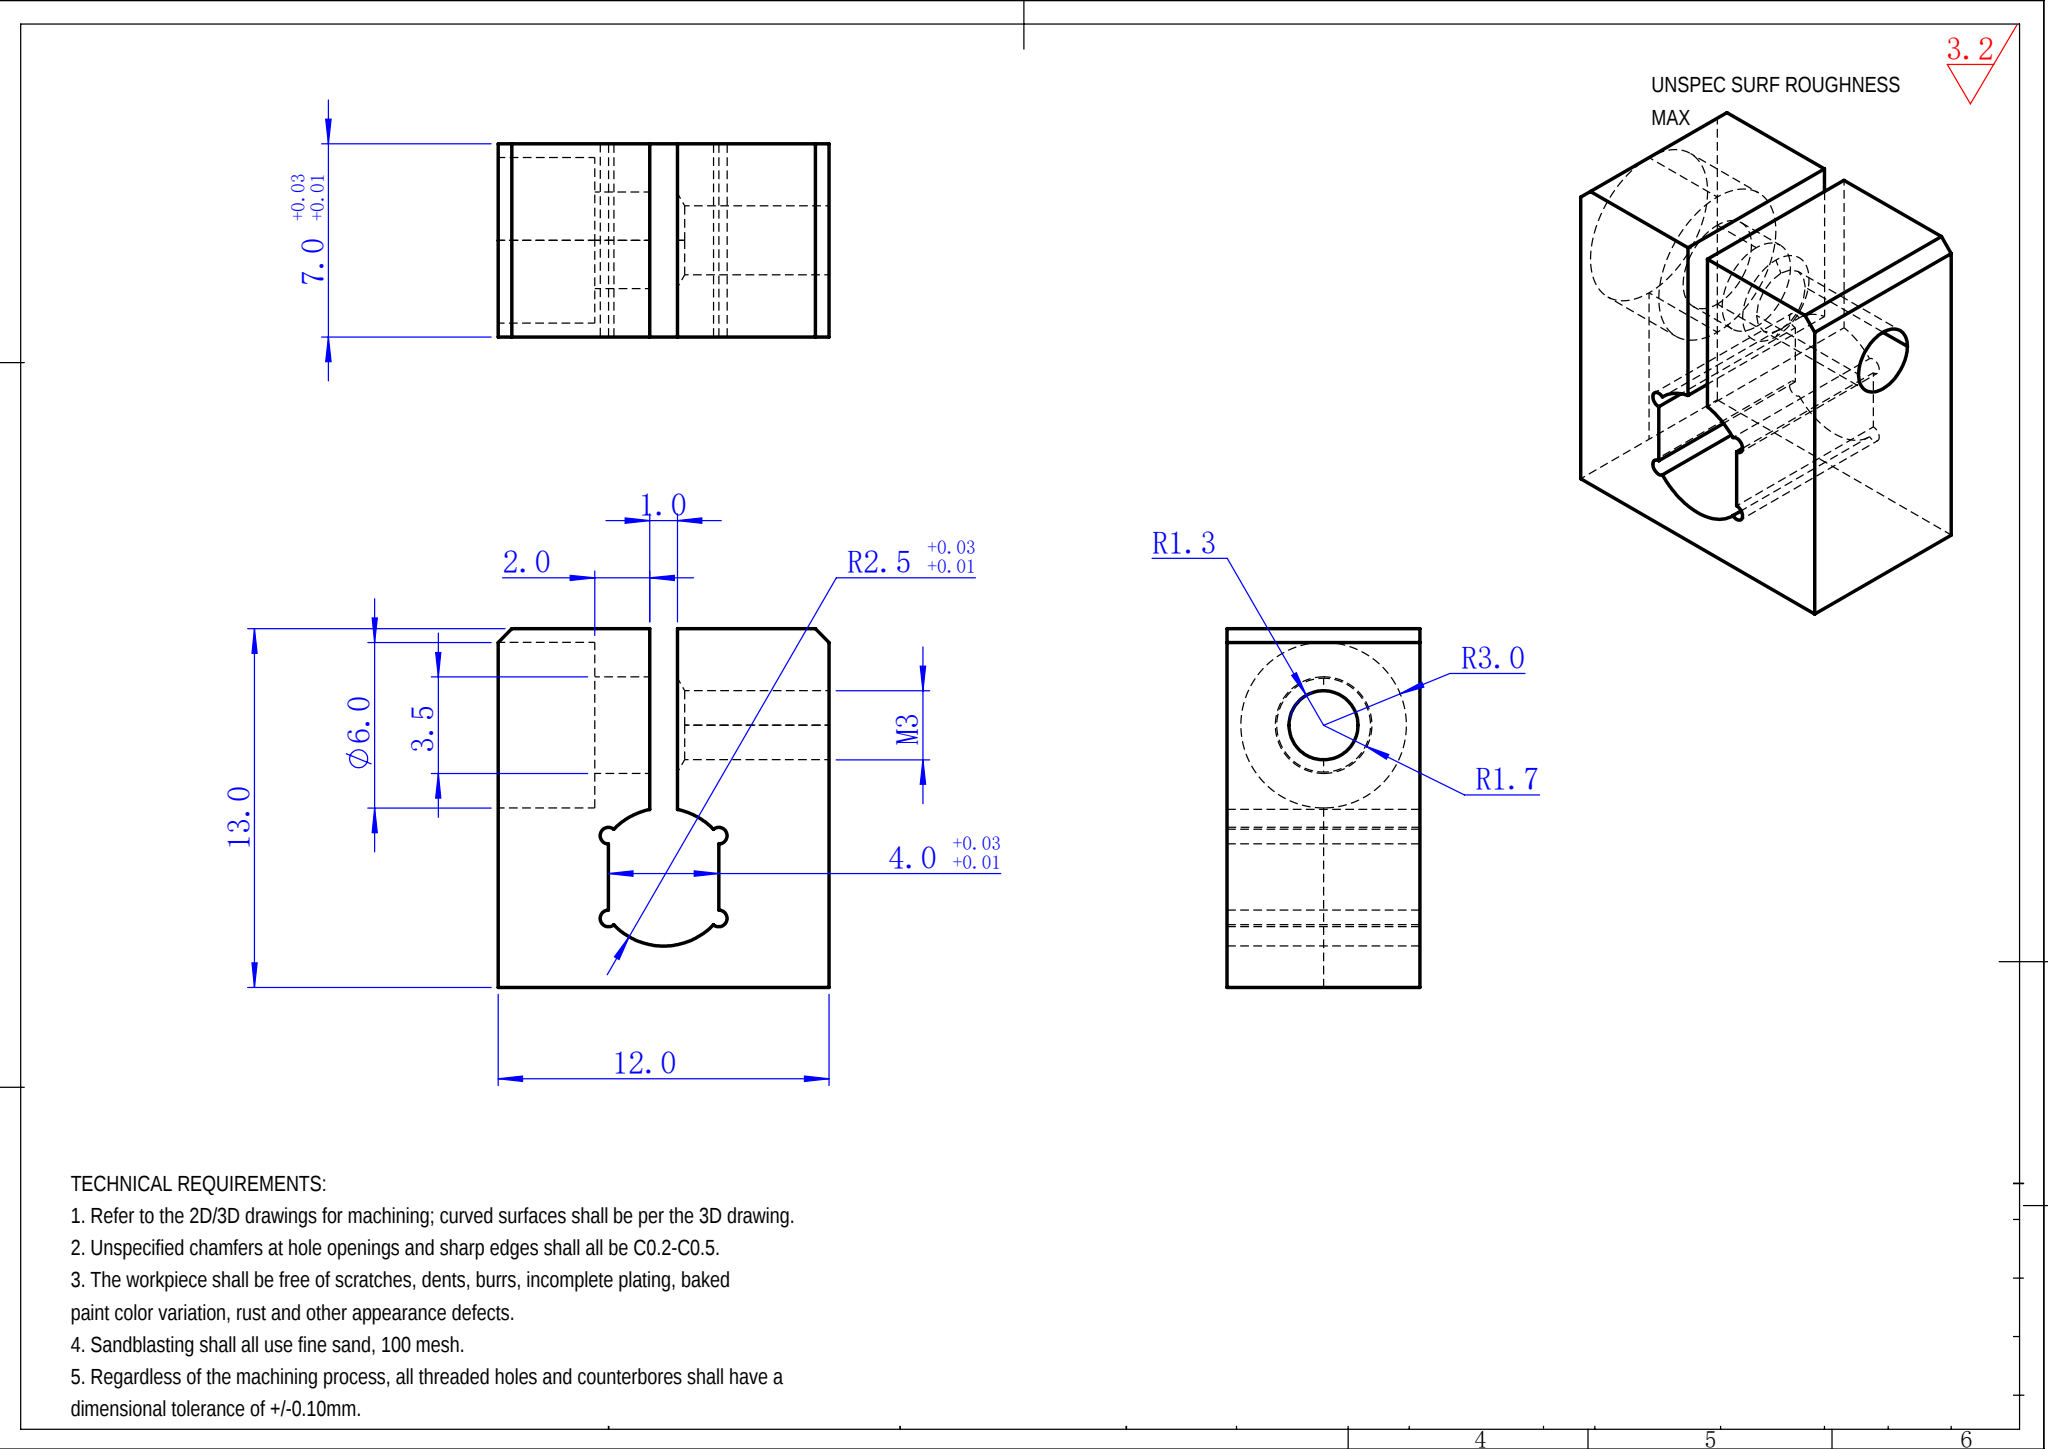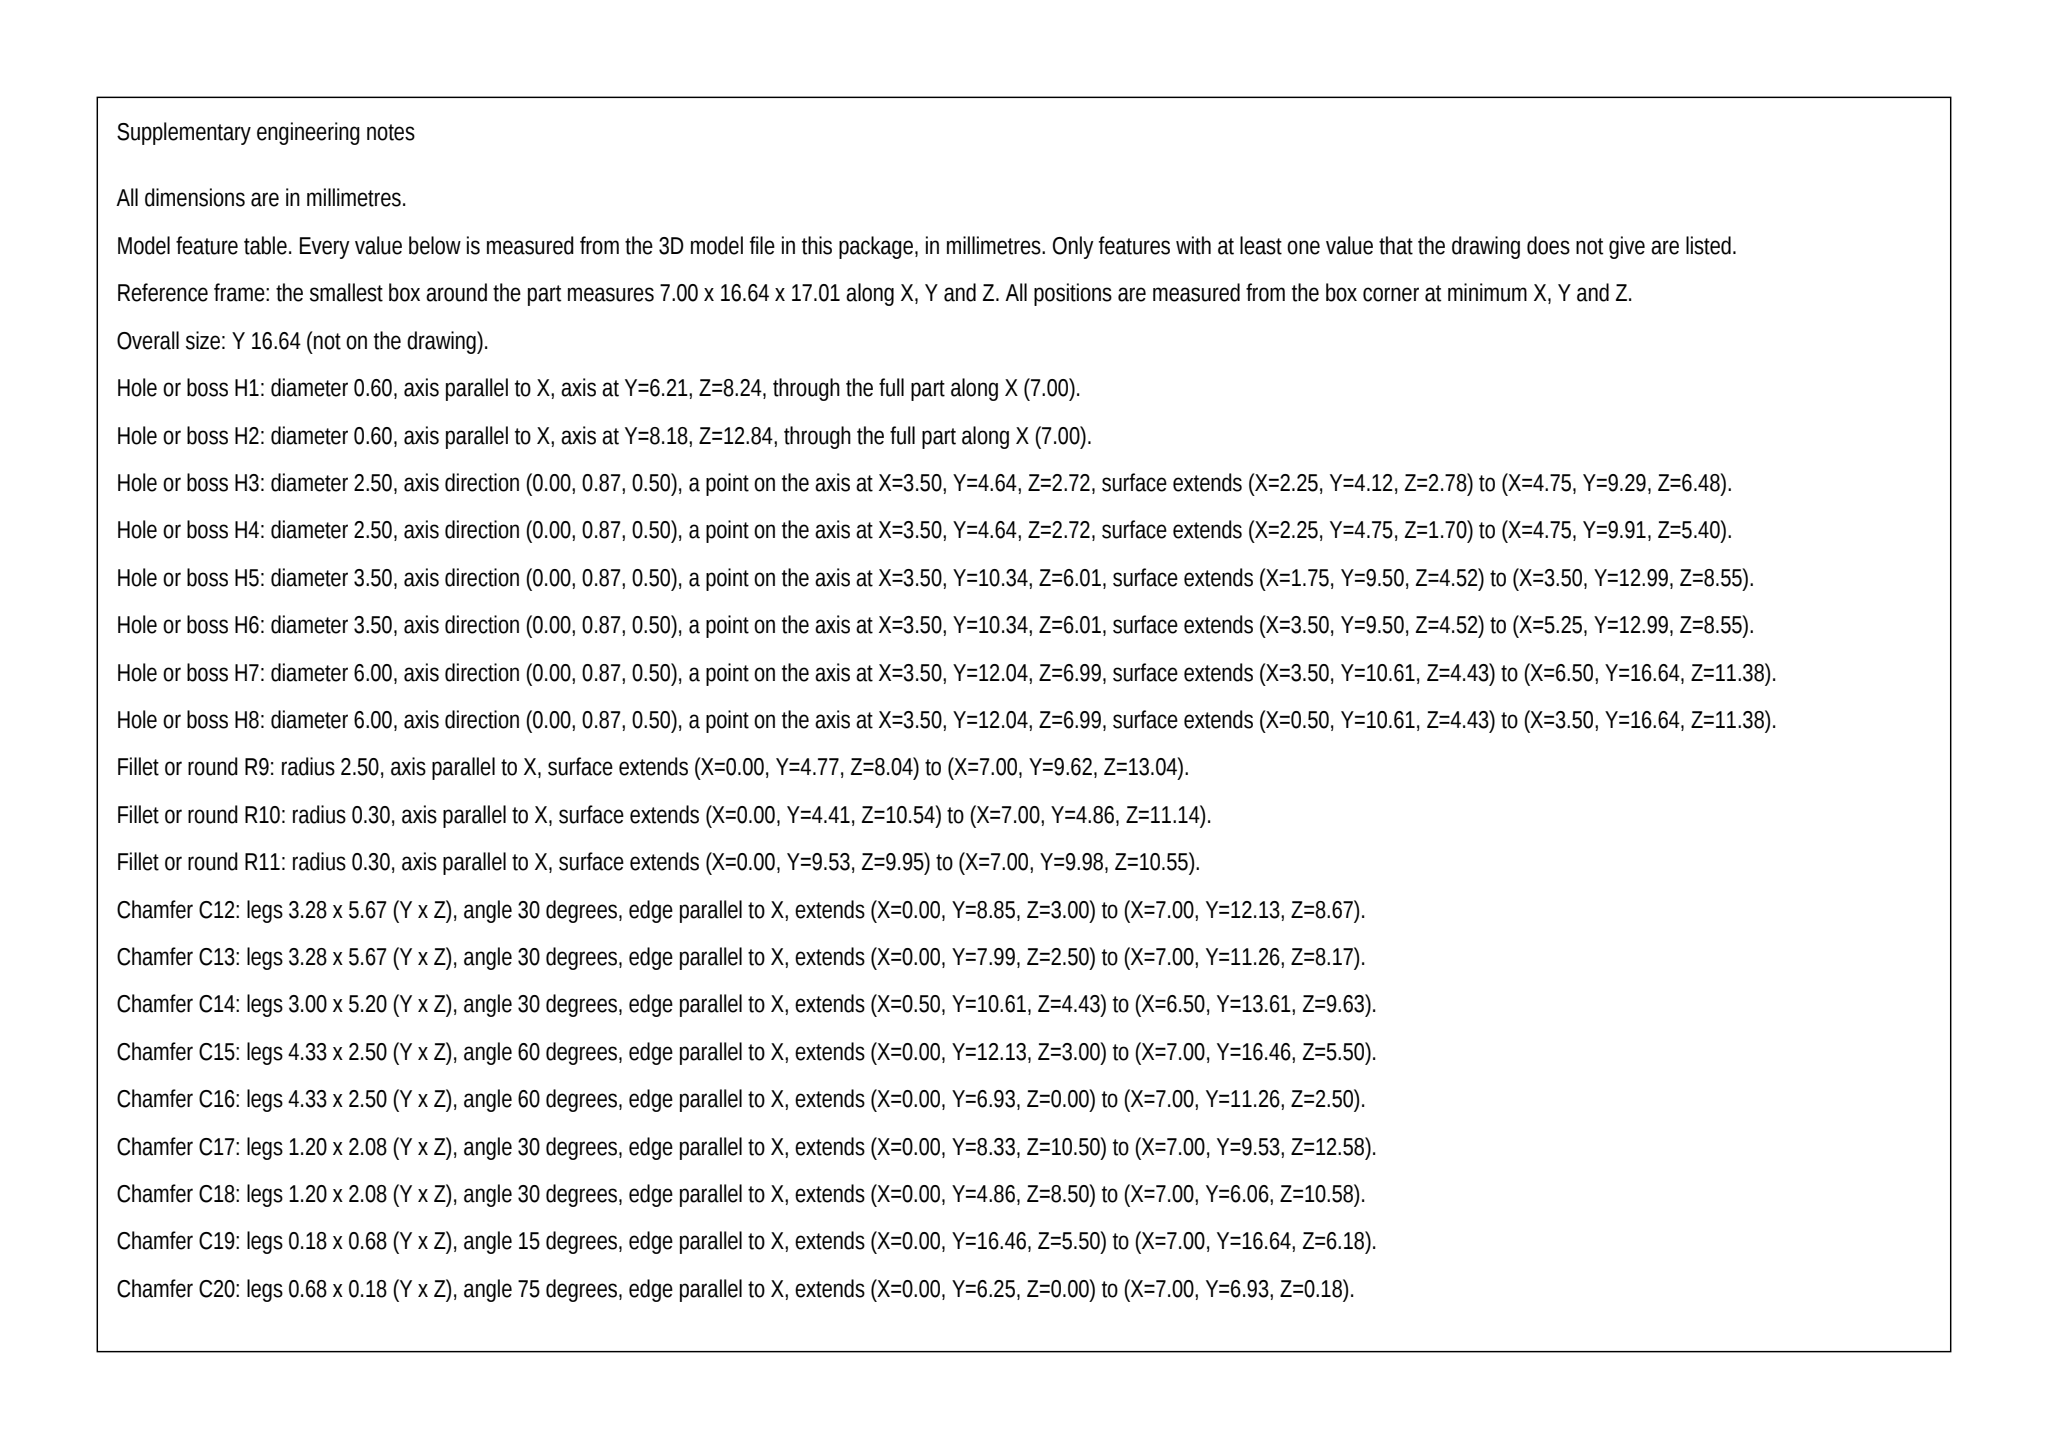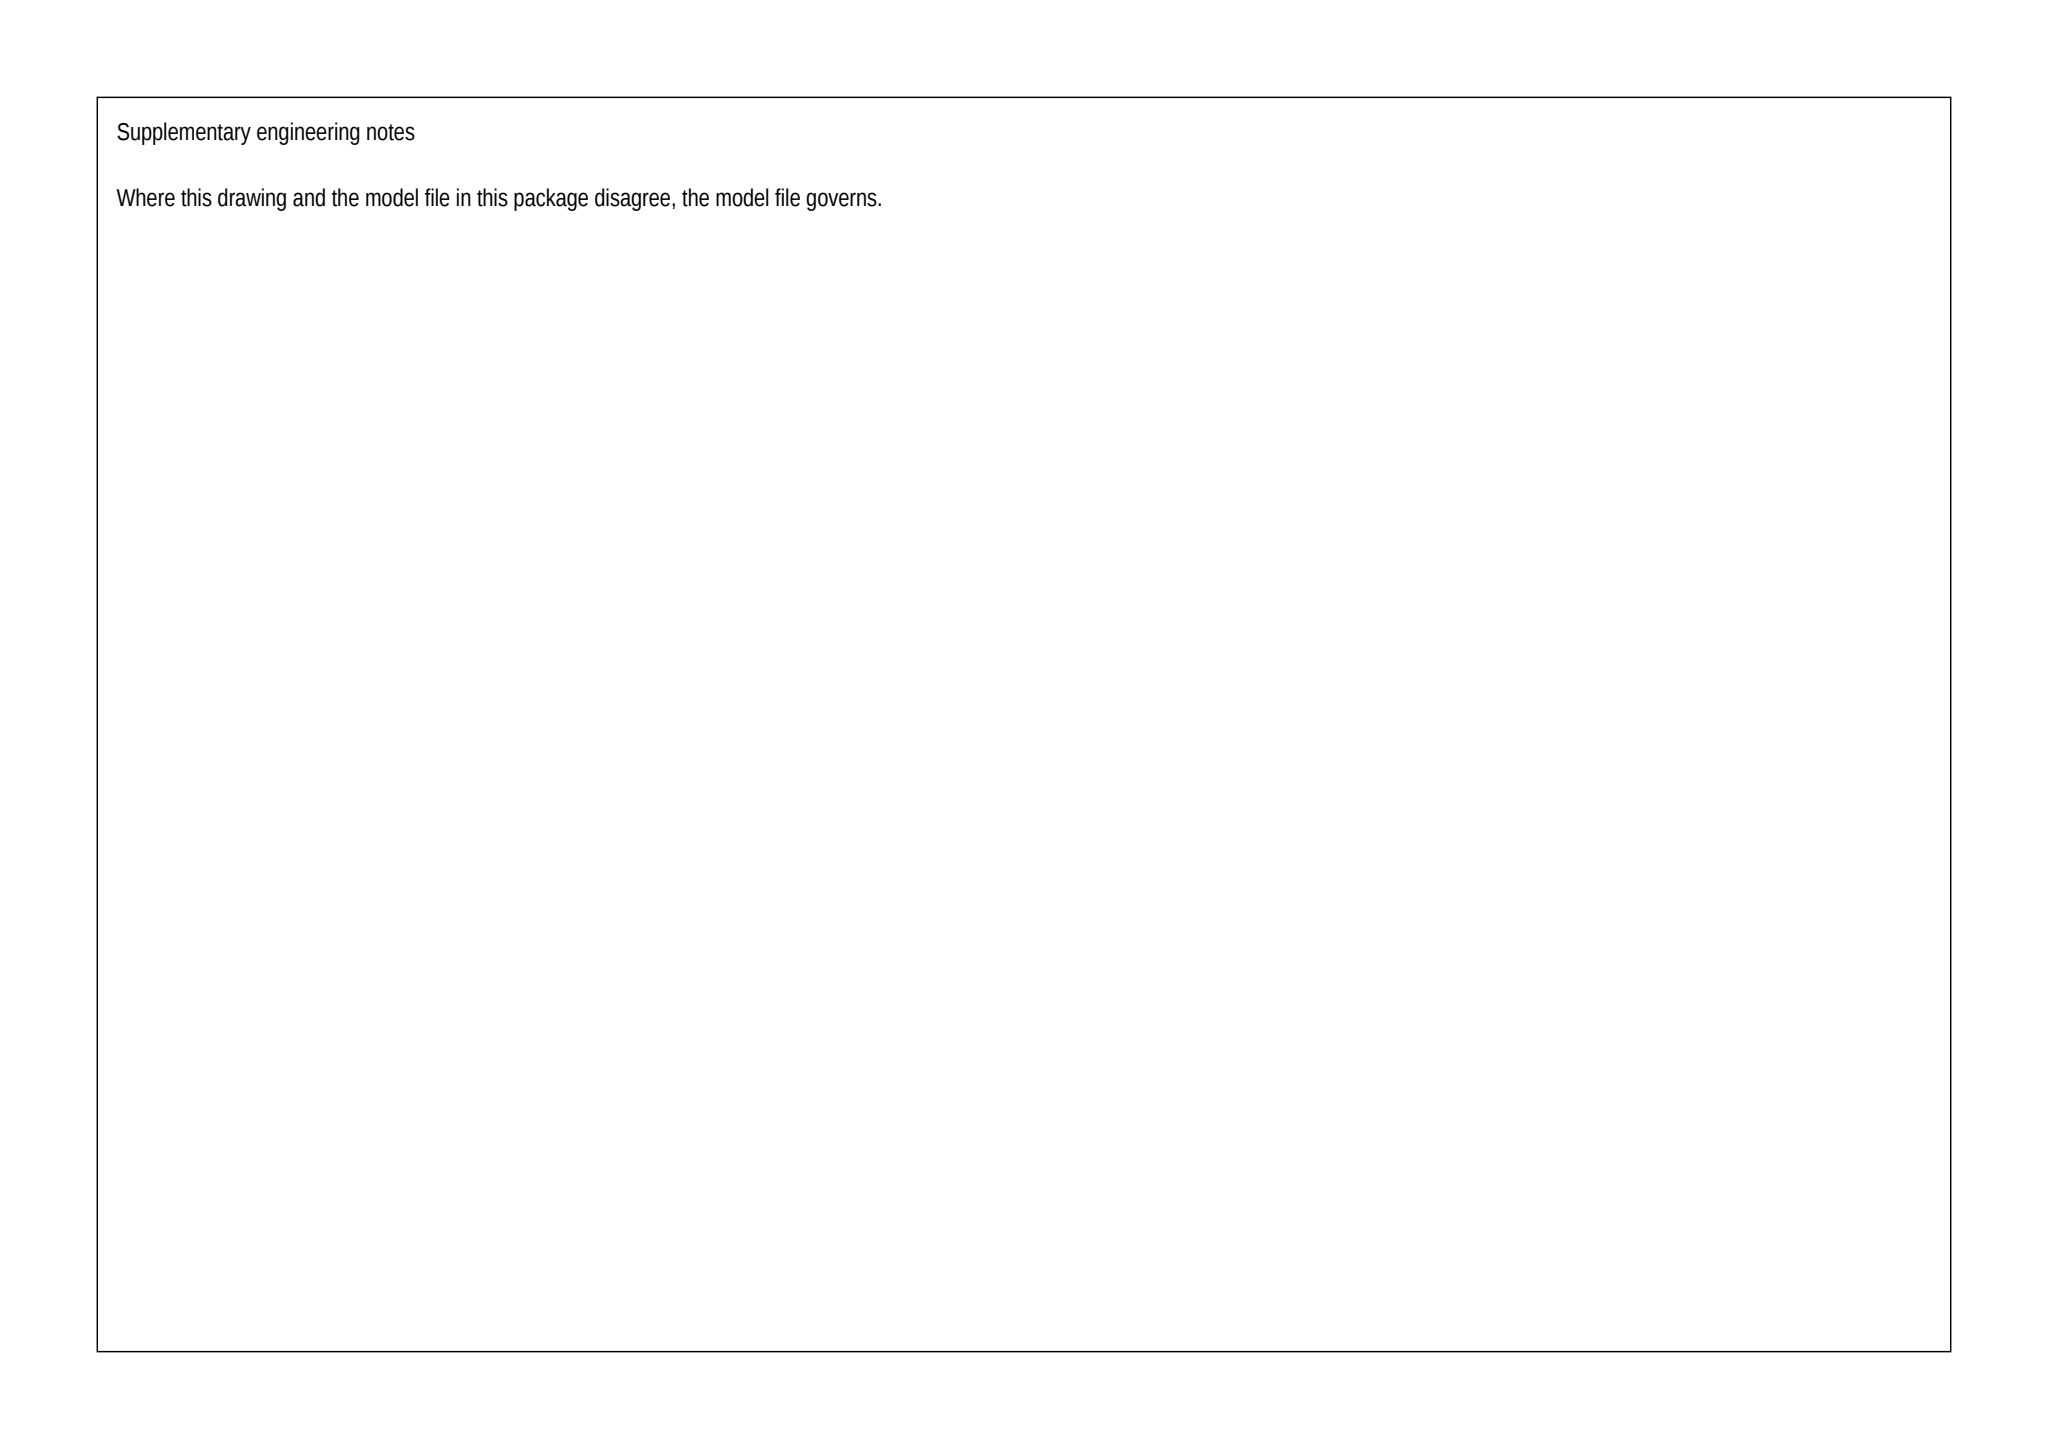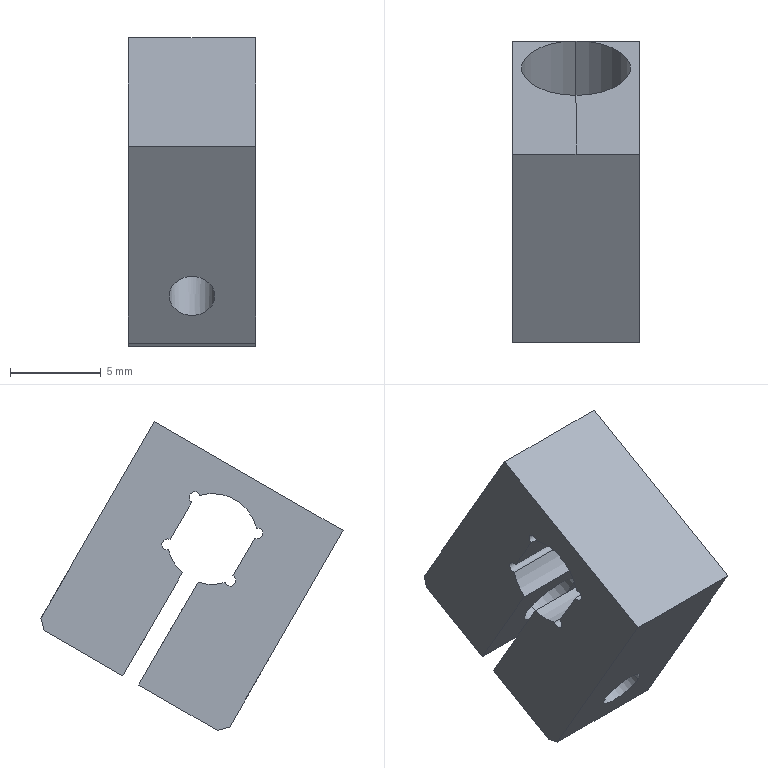Part | SolidWorks | mm | 1 solid | 30 faces | box 7 x 16.64 x 17.01 mm | volume 771 mm3 | plane 15 | cylinder 13 | cone 2 | commonest cylinder face diameters 0.6 x4 5 x3 2.5 x2 3.5 x2 6 x2